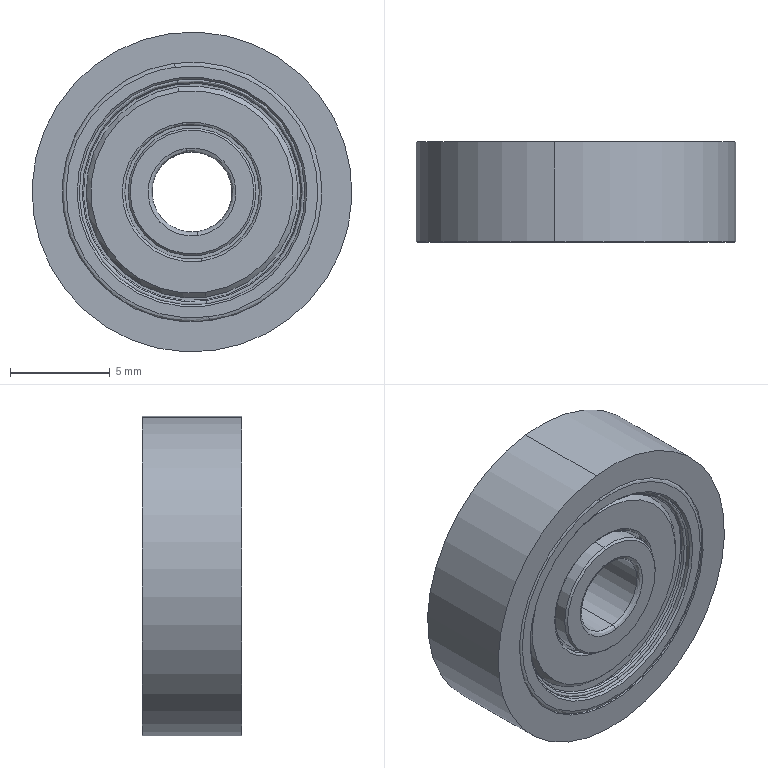Component | SolidWorks | CoatedBearingMisumiUMBGW4-16-1 | 1 solid | 118 faces | volume 785 mm3 | cone 40 | cylinder 32 | spline 28 | plane 18 | commonest cylinder face diameters 13 x4 11.3 x4 6.74 x4 6.973 x4 10.6 x4 7.2 x4 6.4 x4 16 x2 | material 45